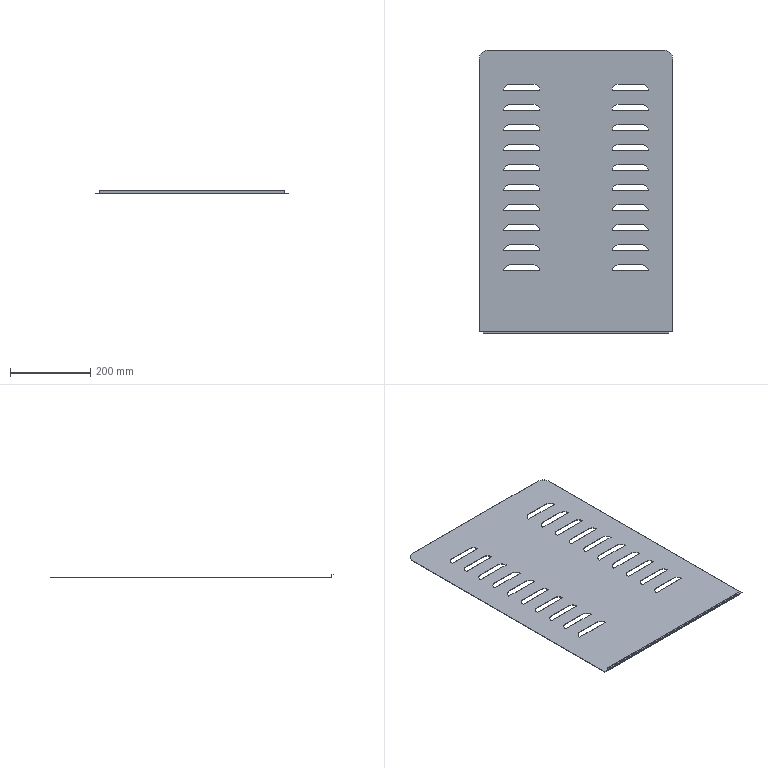Component | SolidWorks | w9-1 | 1 solid | 106 faces | volume 319371 mm3 | plane 60 | cylinder 46 | commonest cylinder face diameters 30 x40 44 x2 3 x2 1 x2